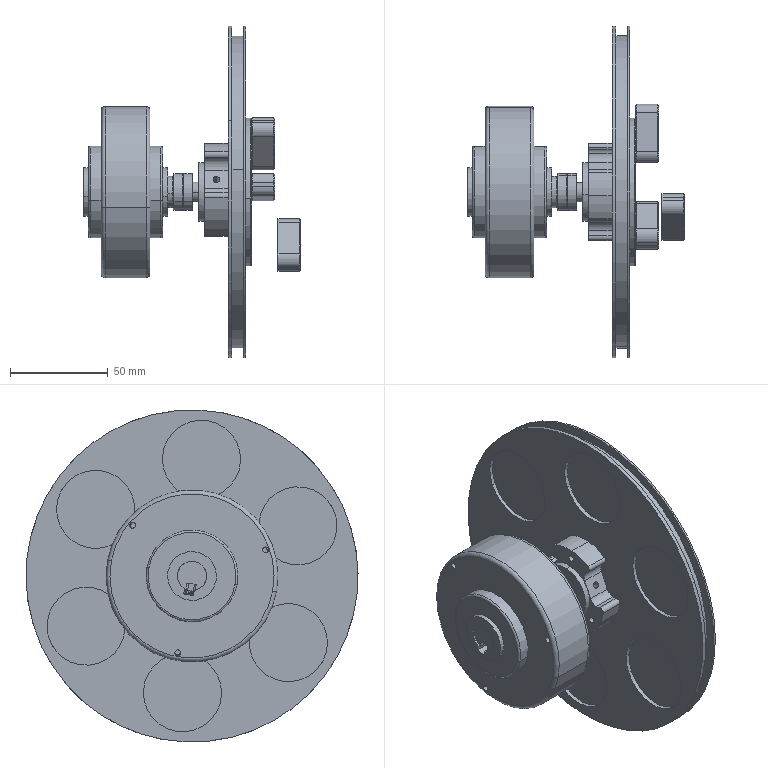Assembly | SolidWorks | mm | 14 component files | 14 solids | 719 faces | box 111.05 x 170 x 170 mm | volume 382199 mm3 | cylinder 227 | sphere 176 | plane 163 | torus 96 | cone 57 | commonest cylinder face diameters 10 x31 3.3 x26 40 x24 17.1 x16 4 x8 13.386 x8 12.6 x8 3 x6
Bill of materials:
2018SOLIDWORKS1000000020 | 1 | 45 Steel | Stepped cylindrical pin/shaft: a longer large-diameter section, a short narrow collar at the step, and a smaller-diameter section whose end face has a small central hole and a slot running from the hole to the outer edge.
2018SOLIDWORKS1000000022 | 1 | 6061 Alloy | Thick circular disc with a central keyed bore, several through-holes spread over the face, and a rectangular notch cut into the outer rim.
2018SOLIDWORKS1000000023 | 3 | 45 Steel | Obround (slot-shaped) block with rounded ends and chamfered edges, with one large central through-hole and two smaller through-holes, one near each end.
2018SOLIDWORKS1000000024 | 1 | 6061 Alloy | Three-lobed hub with a central keyed bore, one axial through-hole in each lobe, concave scalloped cutouts between the lobes, a raised cylindrical boss on one face, and a small radial hole in the outer side.
2018SOLIDWORKS1000000501 | 1 | SKD11 Ejector Pin | Thin flat circular plate with six large circular cutouts around the edge, a small central bore with a key notch, and three small holes around the bore.
2018SOLIDWORKS1000000502 | 1 | 201 | Thin flat annular plate with a large central hole and six circular holes evenly spaced around it.
2018SOLIDWORKS1000000503 | 1 | 201 | Very thin flat ring with a narrow radial width and a large open center.
2018SOLIDWORKS1000000506 | 1 | 201 | Narrow flat ring, slightly thicker than a shim, with a rectangular cross-section and a large open center.
PBT-003 | 1 |  | Wide cylindrical wheel/drum body with rounded outer edges, two-step coaxial hub bosses on both faces, a central keyed bore, and three small holes near the outer edge of the face.
Product-CopperFoilL587-2020 | 1 |  | Thin flat washer-shaped ring with a large central hole.
PurchasedPart_DeepGrooveBallBearing61800-2Z | 2 |  | Ring assembly that looks like a rolling-element bearing: an outer ring and an inner ring with rounded edges, with spherical elements visible in the annular gap between them.
Mates:
1. concentric | 2018SOLIDWORKS1000000022-1 face at (12.716, -108.667, 179.905) dir (1, 0, 0) r 2.1 | 2018SOLIDWORKS1000000023-1 face at (29.769, -108.667, 179.905) dir (1, 0, 0) r 4.5
2. concentric | 2018SOLIDWORKS1000000022-1 face at (12.716, -112.884, 231.696) dir (1, 0, 0) r 2.1 | 2018SOLIDWORKS1000000023-2 face at (16.716, -112.884, 231.696) dir (1, 0, 0) r 4.5
3. concentric | 2018SOLIDWORKS1000000022-1 face at (12.716, -65.924, 209.452) dir (1, 0, 0) r 2.1 | 2018SOLIDWORKS1000000023-3 face at (16.716, -65.924, 209.452) dir (1, 0, 0) r 4.5
4. coincident | 2018SOLIDWORKS1000000022-1 face at (12.716, -95.825, 207.018) dir (1, 0, 0) | 2018SOLIDWORKS1000000023-2 face at (12.716, -112.884, 231.696) dir (-1, 0, 0)
5. coincident | 2018SOLIDWORKS1000000022-1 face at (12.716, -95.825, 207.018) dir (1, 0, 0) | 2018SOLIDWORKS1000000023-3 face at (12.716, -65.924, 209.452) dir (-1, 0, 0)
6. coincident | 2018SOLIDWORKS1000000022-1 face at (2.716, -95.825, 207.018) dir (-1, 0, 0) | 2018SOLIDWORKS1000000501-1 face at (2.716, -95.825, 207.018) dir (1, 0, 0)
7. concentric | 2018SOLIDWORKS1000000022-1 face at (12.716, -95.825, 207.018) dir (-1, 0, 0) r 38 | 2018SOLIDWORKS1000000503-1 face at (7.716, -95.825, 207.018) dir (-1, 0, 0) r 38.25
8. concentric | 2018SOLIDWORKS1000000022-1 face at (12.716, -95.825, 207.018) dir (-1, 0, 0) r 38 | 2018SOLIDWORKS1000000502-1 face at (9.716, -95.825, 207.018) dir (-1, 0, 0) r 38.25
9. coincident | PurchasedPart_DeepGrooveBallBearing61800-2Z-2 face at (-22.284, -98.938, 212.495) dir (1, 0, 0) | PurchasedPart_DeepGrooveBallBearing61800-2Z-1 face at (-22.284, -98.938, 212.495) dir (-1, 0, 0)
10. concentric | 2018SOLIDWORKS1000000022-1 face at (12.716, -95.825, 207.018) dir (-1, 0, 0) r 38 | Product-CopperFoilL587-2020-1 face at (2.716, -95.825, 207.018) dir (1, 0, 0) r 41
11. coincident | 2018SOLIDWORKS1000000501-1 face at (2.716, -95.825, 207.018) dir (1, 0, 0) | Product-CopperFoilL587-2020-1 face at (2.716, -95.825, 207.018) dir (-1, 0, 0)
12. coincident | 2018SOLIDWORKS1000000502-1 face at (8.716, -95.825, 207.018) dir (-1, 0, 0) | Product-CopperFoilL587-2020-1 face at (8.716, -95.825, 207.018) dir (1, 0, 0)
13. concentric | 2018SOLIDWORKS1000000020-1 face at (12.716, -95.825, 207.018) dir (-1, 0, 0) r 5 | 2018SOLIDWORKS1000000024-1 face at (24.758, -95.825, 207.018) dir (-1, 0, 0) r 5
14. concentric | 2018SOLIDWORKS1000000020-1 face at (12.716, -95.825, 207.018) dir (-1, 0, 0) r 5 | PurchasedPart_DeepGrooveBallBearing61800-2Z-1 face at (-19.784, -95.825, 207.018) dir (-1, 0, 0) r 9.5
15. coincident | 2018SOLIDWORKS1000000020-1 face at (-30.284, -95.825, 207.018) dir (-1, 0, 0) | PBT-003-1 face at (-30.284, -95.825, 207.018) dir (1, 0, 0)
16. concentric | 2018SOLIDWORKS1000000020-1 face at (1, -95.825, 207.018) dir (-1, 0, 0) r 7.5 | PBT-003-1 face at (-32.784, -95.825, 207.018) dir (-1, 0, 0) r 7.5
17. concentric | 2018SOLIDWORKS1000000020-1 face at (12.716, -95.825, 207.018) dir (-1, 0, 0) r 5 | 2018SOLIDWORKS1000000022-1 face at (12.716, -95.825, 207.018) dir (-1, 0, 0) r 5
18. concentric | 2018SOLIDWORKS1000000020-1 face at (12.716, -95.825, 207.018) dir (-1, 0, 0) r 5 | 2018SOLIDWORKS1000000501-1 face at (0.7162, -95.825, 207.018) dir (1, 0, 0) r 5.05
19. concentric | 2018SOLIDWORKS1000000020-1 face at (12.716, -95.825, 207.018) dir (-1, 0, 0) r 5 | PurchasedPart_DeepGrooveBallBearing61800-2Z-2 face at (-37.204, -95.825, 207.018) dir (-1, 0, 0) r 5
20. coincident | 2018SOLIDWORKS1000000020-1 face at (-27.284, -95.825, 207.018) dir (1, 0, 0) | PurchasedPart_DeepGrooveBallBearing61800-2Z-2 face at (-27.284, -98.938, 212.495) dir (-1, 0, 0)
21. distance | 2018SOLIDWORKS1000000024-1 face at (-14.284, -95.825, 207.018) dir (-1, 0, 0) | PurchasedPart_DeepGrooveBallBearing61800-2Z-1 face at (-17.284, -98.938, 212.495) dir (1, 0, 0)
22. concentric | 2018SOLIDWORKS1000000022-1 face at (12.716, -77.75, 198.456) dir (1, 0, 0) r 2.15 | 2018SOLIDWORKS1000000501-1 face at (2.716, -77.75, 198.456) dir (1, 0, 0) r 2.25
23. concentric | 2018SOLIDWORKS1000000024-1 face at (-11.284, -77.75, 198.456) dir (-1, 0, 0) r 1.65 | 2018SOLIDWORKS1000000022-1 face at (12.716, -77.75, 198.456) dir (1, 0, 0) r 2.15
24. coincident | 2018SOLIDWORKS1000000024-1 face at (0.7162, -95.825, 207.018) dir (1, 0, 0) | 2018SOLIDWORKS1000000501-1 face at (0.7162, -95.825, 207.018) dir (-1, 0, 0)
25. concentric | 2018SOLIDWORKS1000000022-1 face at (12.716, -95.825, 207.018) dir (-1, 0, 0) r 38 | 2018SOLIDWORKS1000000506-1 face at (6.716, -95.825, 207.018) dir (-1, 0, 0) r 38.25
26. coincident | 2018SOLIDWORKS1000000501-1 face at (2.716, -95.825, 207.018) dir (1, 0, 0) | 2018SOLIDWORKS1000000506-1 face at (2.716, -95.825, 207.018) dir (-1, 0, 0)
27. coincident | 2018SOLIDWORKS1000000503-1 face at (6.716, -95.825, 207.018) dir (-1, 0, 0) | 2018SOLIDWORKS1000000506-1 face at (6.716, -95.825, 207.018) dir (1, 0, 0)